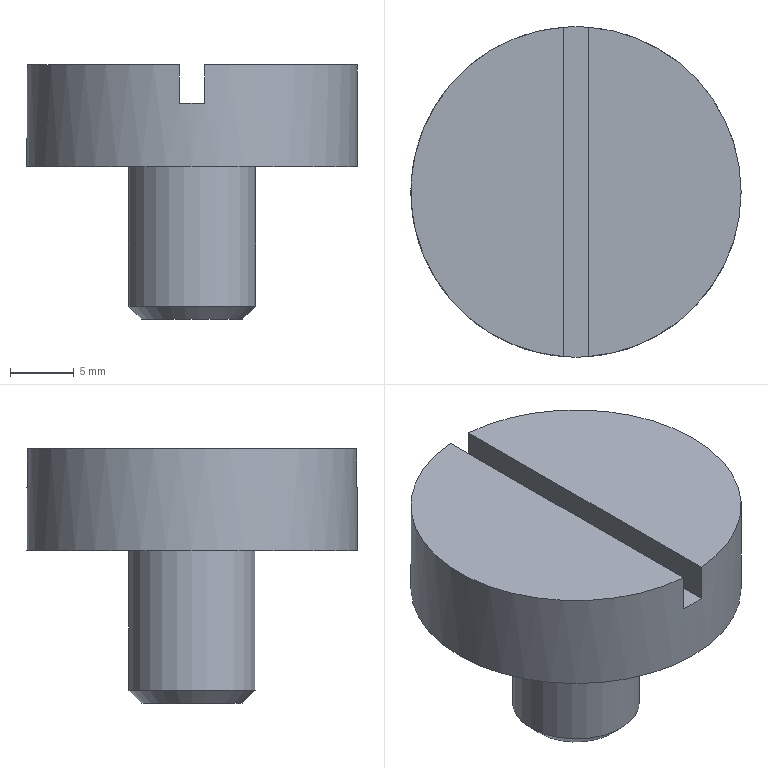Component | NX | 4 | 1 solid | 10 faces | box 26 x 26 x 20 mm | volume 5019 mm3 | plane 7 | cylinder 2 | cone 1 | commonest cylinder face diameters 26 x1 10 x1
STEP:
#1=CARTESIAN_POINT('',(0.,0.,0.));
#2=DIRECTION('',(0.,0.,1.));
#3=DIRECTION('',(1.,0.,0.));
#4=AXIS2_PLACEMENT_3D('',#1,#2,#3);
#5=CARTESIAN_POINT('',(65.,-12.961,57.));
#6=VERTEX_POINT('',#5);
#7=CARTESIAN_POINT('',(65.,12.961,57.));
#8=VERTEX_POINT('',#7);
#9=CARTESIAN_POINT('',(65.,-0.,57.));
#10=DIRECTION('',(0.,1.,0.));
#11=VECTOR('',#10,1.);
#12=LINE('',#9,#11);
#13=CARTESIAN_POINT('',(64.,-0.,57.));
#14=DIRECTION('',(-0.,0.,-1.));
#15=DIRECTION('',(1.,0.,-0.));
#16=AXIS2_PLACEMENT_3D('',#13,#14,#15);
#17=PLANE('',#16);
#18=CARTESIAN_POINT('',(1.,0.));
#19=DIRECTION('',(0.,-1.));
#20=VECTOR('',#19,1.);
#21=LINE('',#18,#20);
#22=(GEOMETRIC_REPRESENTATION_CONTEXT(2)PARAMETRIC_REPRESENTATION_CONTEXT()REPRESENTATION_CONTEXT('',''));
#23=DEFINITIONAL_REPRESENTATION('',(#21),#22);
#24=PCURVE('',#17,#23);
#25=CARTESIAN_POINT('',(65.,-29.5,54.));
#26=DIRECTION('',(-1.,0.,-0.));
#27=DIRECTION('',(0.,0.,-1.));
#28=AXIS2_PLACEMENT_3D('',#25,#26,#27);
#29=PLANE('',#28);
#30=CARTESIAN_POINT('',(-3.,-29.5));
#31=DIRECTION('',(0.,-1.));
#32=VECTOR('',#31,1.);
#33=LINE('',#30,#32);
#34=(GEOMETRIC_REPRESENTATION_CONTEXT(2)PARAMETRIC_REPRESENTATION_CONTEXT()REPRESENTATION_CONTEXT('',''));
#35=DEFINITIONAL_REPRESENTATION('',(#33),#34);
#36=PCURVE('',#29,#35);
#37=SURFACE_CURVE('',#12,(#24,#36),.PCURVE_S1.);
#38=EDGE_CURVE('',#6,#8,#37,.T.);
#39=ORIENTED_EDGE('',*,*,#38,.F.);
#40=CARTESIAN_POINT('',(77.,-0.,57.));
#41=VERTEX_POINT('',#40);
#42=CARTESIAN_POINT('',(64.,-0.,57.));
#43=DIRECTION('',(-0.,0.,-1.));
#44=DIRECTION('',(1.,0.,-0.));
#45=AXIS2_PLACEMENT_3D('',#42,#43,#44);
#46=CIRCLE('',#45,13.);
#47=CARTESIAN_POINT('',(0.,0.));
#48=DIRECTION('',(1.,0.));
#49=AXIS2_PLACEMENT_2D('',#47,#48);
#50=CIRCLE('',#49,13.);
#51=(GEOMETRIC_REPRESENTATION_CONTEXT(2)PARAMETRIC_REPRESENTATION_CONTEXT()REPRESENTATION_CONTEXT('',''));
#52=DEFINITIONAL_REPRESENTATION('',(#50),#51);
#53=PCURVE('',#17,#52);
#54=CARTESIAN_POINT('',(64.,-0.,57.));
#55=DIRECTION('',(-0.,0.,-1.));
#56=DIRECTION('',(1.,0.,-0.));
#57=AXIS2_PLACEMENT_3D('',#54,#55,#56);
#58=CYLINDRICAL_SURFACE('',#57,13.);
#59=CARTESIAN_POINT('',(-6.283,0.));
#60=DIRECTION('',(1.,0.));
#61=VECTOR('',#60,1.);
#62=LINE('',#59,#61);
#63=(GEOMETRIC_REPRESENTATION_CONTEXT(2)PARAMETRIC_REPRESENTATION_CONTEXT()REPRESENTATION_CONTEXT('',''));
#64=DEFINITIONAL_REPRESENTATION('',(#62),#63);
#65=PCURVE('',#58,#64);
#66=SURFACE_CURVE('',#46,(#53,#65),.PCURVE_S1.);
#67=EDGE_CURVE('',#41,#6,#66,.T.);
#68=ORIENTED_EDGE('',*,*,#67,.F.);
#69=CARTESIAN_POINT('',(64.,-0.,57.));
#70=DIRECTION('',(-0.,0.,-1.));
#71=DIRECTION('',(1.,0.,-0.));
#72=AXIS2_PLACEMENT_3D('',#69,#70,#71);
#73=CIRCLE('',#72,13.);
#74=CARTESIAN_POINT('',(0.,0.));
#75=DIRECTION('',(1.,0.));
#76=AXIS2_PLACEMENT_2D('',#74,#75);
#77=CIRCLE('',#76,13.);
#78=(GEOMETRIC_REPRESENTATION_CONTEXT(2)PARAMETRIC_REPRESENTATION_CONTEXT()REPRESENTATION_CONTEXT('',''));
#79=DEFINITIONAL_REPRESENTATION('',(#77),#78);
#80=PCURVE('',#17,#79);
#81=CARTESIAN_POINT('',(0.,0.));
#82=DIRECTION('',(1.,0.));
#83=VECTOR('',#82,1.);
#84=LINE('',#81,#83);
#85=(GEOMETRIC_REPRESENTATION_CONTEXT(2)PARAMETRIC_REPRESENTATION_CONTEXT()REPRESENTATION_CONTEXT('',''));
#86=DEFINITIONAL_REPRESENTATION('',(#84),#85);
#87=PCURVE('',#58,#86);
#88=SURFACE_CURVE('',#73,(#80,#87),.PCURVE_S1.);
#89=EDGE_CURVE('',#8,#41,#88,.T.);
#90=ORIENTED_EDGE('',*,*,#89,.F.);
#91=EDGE_LOOP('',(#39,#68,#90));
#92=FACE_BOUND('',#91,.T.);
#93=ADVANCED_FACE('',(#92),#17,.F.);
#94=CARTESIAN_POINT('',(63.,12.961,57.));
#95=VERTEX_POINT('',#94);
#96=CARTESIAN_POINT('',(63.,-12.961,57.));
#97=VERTEX_POINT('',#96);
#98=CARTESIAN_POINT('',(63.,-0.,57.));
#99=DIRECTION('',(0.,-1.,0.));
#100=VECTOR('',#99,1.);
#101=LINE('',#98,#100);
#102=CARTESIAN_POINT('',(64.,-0.,57.));
#103=DIRECTION('',(-0.,0.,-1.));
#104=DIRECTION('',(1.,0.,-0.));
#105=AXIS2_PLACEMENT_3D('',#102,#103,#104);
#106=PLANE('',#105);
#107=CARTESIAN_POINT('',(-1.,0.));
#108=DIRECTION('',(0.,1.));
#109=VECTOR('',#108,1.);
#110=LINE('',#107,#109);
#111=(GEOMETRIC_REPRESENTATION_CONTEXT(2)PARAMETRIC_REPRESENTATION_CONTEXT()REPRESENTATION_CONTEXT('',''));
#112=DEFINITIONAL_REPRESENTATION('',(#110),#111);
#113=PCURVE('',#106,#112);
#114=CARTESIAN_POINT('',(63.,-29.5,64.278));
#115=DIRECTION('',(1.,0.,-0.));
#116=DIRECTION('',(0.,0.,1.));
#117=AXIS2_PLACEMENT_3D('',#114,#115,#116);
#118=PLANE('',#117);
#119=CARTESIAN_POINT('',(-7.278,-29.5));
#120=DIRECTION('',(0.,1.));
#121=VECTOR('',#120,1.);
#122=LINE('',#119,#121);
#123=(GEOMETRIC_REPRESENTATION_CONTEXT(2)PARAMETRIC_REPRESENTATION_CONTEXT()REPRESENTATION_CONTEXT('',''));
#124=DEFINITIONAL_REPRESENTATION('',(#122),#123);
#125=PCURVE('',#118,#124);
#126=SURFACE_CURVE('',#101,(#113,#125),.PCURVE_S1.);
#127=EDGE_CURVE('',#95,#97,#126,.T.);
#128=ORIENTED_EDGE('',*,*,#127,.F.);
#129=CARTESIAN_POINT('',(64.,-0.,57.));
#130=DIRECTION('',(-0.,0.,-1.));
#131=DIRECTION('',(1.,0.,-0.));
#132=AXIS2_PLACEMENT_3D('',#129,#130,#131);
#133=CIRCLE('',#132,13.);
#134=CARTESIAN_POINT('',(0.,0.));
#135=DIRECTION('',(1.,0.));
#136=AXIS2_PLACEMENT_2D('',#134,#135);
#137=CIRCLE('',#136,13.);
#138=(GEOMETRIC_REPRESENTATION_CONTEXT(2)PARAMETRIC_REPRESENTATION_CONTEXT()REPRESENTATION_CONTEXT('',''));
#139=DEFINITIONAL_REPRESENTATION('',(#137),#138);
#140=PCURVE('',#106,#139);
#141=CARTESIAN_POINT('',(0.,0.));
#142=DIRECTION('',(1.,0.));
#143=VECTOR('',#142,1.);
#144=LINE('',#141,#143);
#145=(GEOMETRIC_REPRESENTATION_CONTEXT(2)PARAMETRIC_REPRESENTATION_CONTEXT()REPRESENTATION_CONTEXT('',''));
#146=DEFINITIONAL_REPRESENTATION('',(#144),#145);
#147=PCURVE('',#58,#146);
#148=SURFACE_CURVE('',#133,(#140,#147),.PCURVE_S1.);
#149=EDGE_CURVE('',#97,#95,#148,.T.);
#150=ORIENTED_EDGE('',*,*,#149,.F.);
#151=EDGE_LOOP('',(#128,#150));
#152=FACE_BOUND('',#151,.T.);
#153=ADVANCED_FACE('',(#152),#106,.F.);
#154=CARTESIAN_POINT('',(77.,-0.,49.));
#155=VERTEX_POINT('',#154);
#156=CARTESIAN_POINT('',(64.,-0.,49.));
#157=DIRECTION('',(-0.,0.,-1.));
#158=DIRECTION('',(1.,0.,-0.));
#159=AXIS2_PLACEMENT_3D('',#156,#157,#158);
#160=CIRCLE('',#159,13.);
#161=CARTESIAN_POINT('',(0.,8.));
#162=DIRECTION('',(1.,0.));
#163=VECTOR('',#162,1.);
#164=LINE('',#161,#163);
#165=(GEOMETRIC_REPRESENTATION_CONTEXT(2)PARAMETRIC_REPRESENTATION_CONTEXT()REPRESENTATION_CONTEXT('',''));
#166=DEFINITIONAL_REPRESENTATION('',(#164),#165);
#167=PCURVE('',#58,#166);
#168=CARTESIAN_POINT('',(51.,-0.,49.));
#169=DIRECTION('',(0.,0.,1.));
#170=DIRECTION('',(-1.,0.,0.));
#171=AXIS2_PLACEMENT_3D('',#168,#169,#170);
#172=PLANE('',#171);
#173=CARTESIAN_POINT('',(-26.,0.));
#174=CARTESIAN_POINT('',(-26.,22.517));
#175=CARTESIAN_POINT('',(-6.5,11.258));
#176=CARTESIAN_POINT('',(13.,0.));
#177=CARTESIAN_POINT('',(-6.5,-11.258));
#178=CARTESIAN_POINT('',(-26.,-22.517));
#179=CARTESIAN_POINT('',(-26.,0.));
#180=(BOUNDED_CURVE()B_SPLINE_CURVE(2,(#173,#174,#175,#176,#177,#178,#179),.UNSPECIFIED.,.T.,.F.)B_SPLINE_CURVE_WITH_KNOTS((1,2,2,2,2,1),(-2.094,0.,2.094,4.189,6.283,8.378),.UNSPECIFIED.)CURVE()GEOMETRIC_REPRESENTATION_ITEM()RATIONAL_B_SPLINE_CURVE((1.,0.5,1.,0.5,1.,0.5,1.))REPRESENTATION_ITEM(''));
#181=(GEOMETRIC_REPRESENTATION_CONTEXT(2)PARAMETRIC_REPRESENTATION_CONTEXT()REPRESENTATION_CONTEXT('',''));
#182=DEFINITIONAL_REPRESENTATION('',(#180),#181);
#183=PCURVE('',#172,#182);
#184=SURFACE_CURVE('',#160,(#167,#183),.PCURVE_S1.);
#185=EDGE_CURVE('',#155,#155,#184,.T.);
#186=ORIENTED_EDGE('',*,*,#185,.F.);
#187=CARTESIAN_POINT('',(77.,-0.,57.));
#188=CARTESIAN_POINT('',(77.,-0.,49.));
#189=B_SPLINE_CURVE_WITH_KNOTS('',1,(#187,#188),.UNSPECIFIED.,.F.,.F.,(2,2),(0.,8.),.PIECEWISE_BEZIER_KNOTS.);
#190=CARTESIAN_POINT('',(0.,0.));
#191=DIRECTION('',(0.,1.));
#192=VECTOR('',#191,1.);
#193=LINE('',#190,#192);
#194=(GEOMETRIC_REPRESENTATION_CONTEXT(2)PARAMETRIC_REPRESENTATION_CONTEXT()REPRESENTATION_CONTEXT('',''));
#195=DEFINITIONAL_REPRESENTATION('',(#193),#194);
#196=PCURVE('',#58,#195);
#197=CARTESIAN_POINT('',(6.283,0.));
#198=DIRECTION('',(0.,1.));
#199=VECTOR('',#198,1.);
#200=LINE('',#197,#199);
#201=(GEOMETRIC_REPRESENTATION_CONTEXT(2)PARAMETRIC_REPRESENTATION_CONTEXT()REPRESENTATION_CONTEXT('',''));
#202=DEFINITIONAL_REPRESENTATION('',(#200),#201);
#203=PCURVE('',#58,#202);
#204=SEAM_CURVE('',#189,(#196,#203),.PCURVE_S1.);
#205=EDGE_CURVE('',#41,#155,#204,.T.);
#206=ORIENTED_EDGE('',*,*,#205,.F.);
#207=ORIENTED_EDGE('',*,*,#67,.T.);
#208=CARTESIAN_POINT('',(65.,-12.961,54.));
#209=VERTEX_POINT('',#208);
#210=CARTESIAN_POINT('',(65.,-12.961,57.));
#211=DIRECTION('',(0.,0.,1.));
#212=VECTOR('',#211,1.);
#213=LINE('',#210,#212);
#214=CARTESIAN_POINT('',(1.494,0.));
#215=DIRECTION('',(0.,-1.));
#216=VECTOR('',#215,1.);
#217=LINE('',#214,#216);
#218=(GEOMETRIC_REPRESENTATION_CONTEXT(2)PARAMETRIC_REPRESENTATION_CONTEXT()REPRESENTATION_CONTEXT('',''));
#219=DEFINITIONAL_REPRESENTATION('',(#217),#218);
#220=PCURVE('',#58,#219);
#221=CARTESIAN_POINT('',(-3.,-16.539));
#222=DIRECTION('',(-1.,0.));
#223=VECTOR('',#222,1.);
#224=LINE('',#221,#223);
#225=(GEOMETRIC_REPRESENTATION_CONTEXT(2)PARAMETRIC_REPRESENTATION_CONTEXT()REPRESENTATION_CONTEXT('',''));
#226=DEFINITIONAL_REPRESENTATION('',(#224),#225);
#227=PCURVE('',#29,#226);
#228=SURFACE_CURVE('',#213,(#220,#227),.PCURVE_S1.);
#229=EDGE_CURVE('',#209,#6,#228,.T.);
#230=ORIENTED_EDGE('',*,*,#229,.F.);
#231=CARTESIAN_POINT('',(63.,-12.961,54.));
#232=VERTEX_POINT('',#231);
#233=CARTESIAN_POINT('',(64.,-0.,54.));
#234=DIRECTION('',(0.,0.,1.));
#235=DIRECTION('',(-1.,0.,0.));
#236=AXIS2_PLACEMENT_3D('',#233,#234,#235);
#237=CIRCLE('',#236,13.);
#238=CARTESIAN_POINT('',(3.142,3.));
#239=DIRECTION('',(-1.,0.));
#240=VECTOR('',#239,1.);
#241=LINE('',#238,#240);
#242=(GEOMETRIC_REPRESENTATION_CONTEXT(2)PARAMETRIC_REPRESENTATION_CONTEXT()REPRESENTATION_CONTEXT('',''));
#243=DEFINITIONAL_REPRESENTATION('',(#241),#242);
#244=PCURVE('',#58,#243);
#245=CARTESIAN_POINT('',(63.,-29.5,54.));
#246=DIRECTION('',(0.,0.,1.));
#247=DIRECTION('',(-1.,0.,0.));
#248=AXIS2_PLACEMENT_3D('',#245,#246,#247);
#249=PLANE('',#248);
#250=CARTESIAN_POINT('',(-1.,-29.5));
#251=DIRECTION('',(1.,0.));
#252=AXIS2_PLACEMENT_2D('',#250,#251);
#253=CIRCLE('',#252,13.);
#254=(GEOMETRIC_REPRESENTATION_CONTEXT(2)PARAMETRIC_REPRESENTATION_CONTEXT()REPRESENTATION_CONTEXT('',''));
#255=DEFINITIONAL_REPRESENTATION('',(#253),#254);
#256=PCURVE('',#249,#255);
#257=SURFACE_CURVE('',#237,(#244,#256),.PCURVE_S1.);
#258=EDGE_CURVE('',#232,#209,#257,.T.);
#259=ORIENTED_EDGE('',*,*,#258,.F.);
#260=CARTESIAN_POINT('',(63.,-12.961,57.));
#261=DIRECTION('',(-0.,0.,-1.));
#262=VECTOR('',#261,1.);
#263=LINE('',#260,#262);
#264=CARTESIAN_POINT('',(1.648,0.));
#265=DIRECTION('',(-0.,1.));
#266=VECTOR('',#265,1.);
#267=LINE('',#264,#266);
#268=(GEOMETRIC_REPRESENTATION_CONTEXT(2)PARAMETRIC_REPRESENTATION_CONTEXT()REPRESENTATION_CONTEXT('',''));
#269=DEFINITIONAL_REPRESENTATION('',(#267),#268);
#270=PCURVE('',#58,#269);
#271=CARTESIAN_POINT('',(-7.278,-16.539));
#272=DIRECTION('',(-1.,0.));
#273=VECTOR('',#272,1.);
#274=LINE('',#271,#273);
#275=(GEOMETRIC_REPRESENTATION_CONTEXT(2)PARAMETRIC_REPRESENTATION_CONTEXT()REPRESENTATION_CONTEXT('',''));
#276=DEFINITIONAL_REPRESENTATION('',(#274),#275);
#277=PCURVE('',#118,#276);
#278=SURFACE_CURVE('',#263,(#270,#277),.PCURVE_S1.);
#279=EDGE_CURVE('',#97,#232,#278,.T.);
#280=ORIENTED_EDGE('',*,*,#279,.F.);
#281=ORIENTED_EDGE('',*,*,#149,.T.);
#282=CARTESIAN_POINT('',(63.,12.961,54.));
#283=VERTEX_POINT('',#282);
#284=CARTESIAN_POINT('',(63.,12.961,57.));
#285=DIRECTION('',(0.,0.,1.));
#286=VECTOR('',#285,1.);
#287=LINE('',#284,#286);
#288=CARTESIAN_POINT('',(4.635,0.));
#289=DIRECTION('',(-0.,-1.));
#290=VECTOR('',#289,1.);
#291=LINE('',#288,#290);
#292=(GEOMETRIC_REPRESENTATION_CONTEXT(2)PARAMETRIC_REPRESENTATION_CONTEXT()REPRESENTATION_CONTEXT('',''));
#293=DEFINITIONAL_REPRESENTATION('',(#291),#292);
#294=PCURVE('',#58,#293);
#295=CARTESIAN_POINT('',(-7.278,-42.461));
#296=DIRECTION('',(1.,0.));
#297=VECTOR('',#296,1.);
#298=LINE('',#295,#297);
#299=(GEOMETRIC_REPRESENTATION_CONTEXT(2)PARAMETRIC_REPRESENTATION_CONTEXT()REPRESENTATION_CONTEXT('',''));
#300=DEFINITIONAL_REPRESENTATION('',(#298),#299);
#301=PCURVE('',#118,#300);
#302=SURFACE_CURVE('',#287,(#294,#301),.PCURVE_S1.);
#303=EDGE_CURVE('',#283,#95,#302,.T.);
#304=ORIENTED_EDGE('',*,*,#303,.F.);
#305=CARTESIAN_POINT('',(65.,12.961,54.));
#306=VERTEX_POINT('',#305);
#307=CARTESIAN_POINT('',(64.,-0.,54.));
#308=DIRECTION('',(0.,0.,1.));
#309=DIRECTION('',(-1.,0.,0.));
#310=AXIS2_PLACEMENT_3D('',#307,#308,#309);
#311=CIRCLE('',#310,13.);
#312=CARTESIAN_POINT('',(9.425,3.));
#313=DIRECTION('',(-1.,0.));
#314=VECTOR('',#313,1.);
#315=LINE('',#312,#314);
#316=(GEOMETRIC_REPRESENTATION_CONTEXT(2)PARAMETRIC_REPRESENTATION_CONTEXT()REPRESENTATION_CONTEXT('',''));
#317=DEFINITIONAL_REPRESENTATION('',(#315),#316);
#318=PCURVE('',#58,#317);
#319=CARTESIAN_POINT('',(-1.,-29.5));
#320=DIRECTION('',(1.,0.));
#321=AXIS2_PLACEMENT_2D('',#319,#320);
#322=CIRCLE('',#321,13.);
#323=(GEOMETRIC_REPRESENTATION_CONTEXT(2)PARAMETRIC_REPRESENTATION_CONTEXT()REPRESENTATION_CONTEXT('',''));
#324=DEFINITIONAL_REPRESENTATION('',(#322),#323);
#325=PCURVE('',#249,#324);
#326=SURFACE_CURVE('',#311,(#318,#325),.PCURVE_S1.);
#327=EDGE_CURVE('',#306,#283,#326,.T.);
#328=ORIENTED_EDGE('',*,*,#327,.F.);
#329=CARTESIAN_POINT('',(65.,12.961,57.));
#330=DIRECTION('',(-0.,0.,-1.));
#331=VECTOR('',#330,1.);
#332=LINE('',#329,#331);
#333=CARTESIAN_POINT('',(4.789,0.));
#334=DIRECTION('',(0.,1.));
#335=VECTOR('',#334,1.);
#336=LINE('',#333,#335);
#337=(GEOMETRIC_REPRESENTATION_CONTEXT(2)PARAMETRIC_REPRESENTATION_CONTEXT()REPRESENTATION_CONTEXT('',''));
#338=DEFINITIONAL_REPRESENTATION('',(#336),#337);
#339=PCURVE('',#58,#338);
#340=CARTESIAN_POINT('',(-3.,-42.461));
#341=DIRECTION('',(1.,0.));
#342=VECTOR('',#341,1.);
#343=LINE('',#340,#342);
#344=(GEOMETRIC_REPRESENTATION_CONTEXT(2)PARAMETRIC_REPRESENTATION_CONTEXT()REPRESENTATION_CONTEXT('',''));
#345=DEFINITIONAL_REPRESENTATION('',(#343),#344);
#346=PCURVE('',#29,#345);
#347=SURFACE_CURVE('',#332,(#339,#346),.PCURVE_S1.);
#348=EDGE_CURVE('',#8,#306,#347,.T.);
#349=ORIENTED_EDGE('',*,*,#348,.F.);
#350=ORIENTED_EDGE('',*,*,#89,.T.);
#351=ORIENTED_EDGE('',*,*,#205,.T.);
#352=EDGE_LOOP('',(#186,#206,#207,#230,#259,#280,#281,#304,#328,#349,#350,#351));
#353=FACE_BOUND('',#352,.T.);
#354=ADVANCED_FACE('',(#353),#58,.T.);
#355=CARTESIAN_POINT('',(60.,-0.,37.));
#356=VERTEX_POINT('',#355);
#357=CARTESIAN_POINT('',(64.,-0.,37.));
#358=DIRECTION('',(-0.,0.,-1.));
#359=DIRECTION('',(-1.,0.,0.));
#360=AXIS2_PLACEMENT_3D('',#357,#358,#359);
#361=CIRCLE('',#360,4.);
#362=CARTESIAN_POINT('',(59.,-0.,37.));
#363=DIRECTION('',(0.,0.,1.));
#364=DIRECTION('',(-1.,0.,0.));
#365=AXIS2_PLACEMENT_3D('',#362,#363,#364);
#366=PLANE('',#365);
#367=CARTESIAN_POINT('',(-1.,0.));
#368=CARTESIAN_POINT('',(-1.,-6.928));
#369=CARTESIAN_POINT('',(-7.,-3.464));
#370=CARTESIAN_POINT('',(-13.,-0.));
#371=CARTESIAN_POINT('',(-7.,3.464));
#372=CARTESIAN_POINT('',(-1.,6.928));
#373=CARTESIAN_POINT('',(-1.,0.));
#374=(BOUNDED_CURVE()B_SPLINE_CURVE(2,(#367,#368,#369,#370,#371,#372,#373),.UNSPECIFIED.,.T.,.F.)B_SPLINE_CURVE_WITH_KNOTS((1,2,2,2,2,1),(-2.094,0.,2.094,4.189,6.283,8.378),.UNSPECIFIED.)CURVE()GEOMETRIC_REPRESENTATION_ITEM()RATIONAL_B_SPLINE_CURVE((1.,0.5,1.,0.5,1.,0.5,1.))REPRESENTATION_ITEM(''));
#375=(GEOMETRIC_REPRESENTATION_CONTEXT(2)PARAMETRIC_REPRESENTATION_CONTEXT()REPRESENTATION_CONTEXT('',''));
#376=DEFINITIONAL_REPRESENTATION('',(#374),#375);
#377=PCURVE('',#366,#376);
#378=CARTESIAN_POINT('',(64.,-0.,37.));
#379=DIRECTION('',(0.,0.,1.));
#380=DIRECTION('',(-1.,0.,0.));
#381=AXIS2_PLACEMENT_3D('',#378,#379,#380);
#382=CONICAL_SURFACE('',#381,4.,0.7854);
#383=CARTESIAN_POINT('',(6.283,-0.));
#384=DIRECTION('',(-1.,0.));
#385=VECTOR('',#384,1.);
#386=LINE('',#383,#385);
#387=(GEOMETRIC_REPRESENTATION_CONTEXT(2)PARAMETRIC_REPRESENTATION_CONTEXT()REPRESENTATION_CONTEXT('',''));
#388=DEFINITIONAL_REPRESENTATION('',(#386),#387);
#389=PCURVE('',#382,#388);
#390=SURFACE_CURVE('',#361,(#377,#389),.PCURVE_S1.);
#391=EDGE_CURVE('',#356,#356,#390,.T.);
#392=ORIENTED_EDGE('',*,*,#391,.T.);
#393=EDGE_LOOP('',(#392));
#394=FACE_BOUND('',#393,.T.);
#395=ADVANCED_FACE('',(#394),#366,.F.);
#396=CARTESIAN_POINT('',(69.,-0.,49.));
#397=VERTEX_POINT('',#396);
#398=CARTESIAN_POINT('',(64.,-0.,49.));
#399=DIRECTION('',(-0.,0.,-1.));
#400=DIRECTION('',(1.,0.,-0.));
#401=AXIS2_PLACEMENT_3D('',#398,#399,#400);
#402=CIRCLE('',#401,5.);
#403=CARTESIAN_POINT('',(-18.,0.));
#404=CARTESIAN_POINT('',(-18.,8.66));
#405=CARTESIAN_POINT('',(-10.5,4.33));
#406=CARTESIAN_POINT('',(-3.,0.));
#407=CARTESIAN_POINT('',(-10.5,-4.33));
#408=CARTESIAN_POINT('',(-18.,-8.66));
#409=CARTESIAN_POINT('',(-18.,0.));
#410=(BOUNDED_CURVE()B_SPLINE_CURVE(2,(#403,#404,#405,#406,#407,#408,#409),.UNSPECIFIED.,.T.,.F.)B_SPLINE_CURVE_WITH_KNOTS((1,2,2,2,2,1),(-2.094,0.,2.094,4.189,6.283,8.378),.UNSPECIFIED.)CURVE()GEOMETRIC_REPRESENTATION_ITEM()RATIONAL_B_SPLINE_CURVE((1.,0.5,1.,0.5,1.,0.5,1.))REPRESENTATION_ITEM(''));
#411=(GEOMETRIC_REPRESENTATION_CONTEXT(2)PARAMETRIC_REPRESENTATION_CONTEXT()REPRESENTATION_CONTEXT('',''));
#412=DEFINITIONAL_REPRESENTATION('',(#410),#411);
#413=PCURVE('',#172,#412);
#414=CARTESIAN_POINT('',(64.,-0.,57.));
#415=DIRECTION('',(-0.,0.,-1.));
#416=DIRECTION('',(1.,0.,-0.));
#417=AXIS2_PLACEMENT_3D('',#414,#415,#416);
#418=CYLINDRICAL_SURFACE('',#417,5.);
#419=CARTESIAN_POINT('',(0.,8.));
#420=DIRECTION('',(1.,0.));
#421=VECTOR('',#420,1.);
#422=LINE('',#419,#421);
#423=(GEOMETRIC_REPRESENTATION_CONTEXT(2)PARAMETRIC_REPRESENTATION_CONTEXT()REPRESENTATION_CONTEXT('',''));
#424=DEFINITIONAL_REPRESENTATION('',(#422),#423);
#425=PCURVE('',#418,#424);
#426=SURFACE_CURVE('',#402,(#413,#425),.PCURVE_S1.);
#427=EDGE_CURVE('',#397,#397,#426,.T.);
#428=ORIENTED_EDGE('',*,*,#427,.F.);
#429=EDGE_LOOP('',(#428));
#430=FACE_BOUND('',#429,.T.);
#431=ORIENTED_EDGE('',*,*,#185,.T.);
#432=EDGE_LOOP('',(#431));
#433=FACE_BOUND('',#432,.T.);
#434=ADVANCED_FACE('',(#430,#433),#172,.F.);
#435=CARTESIAN_POINT('',(59.,-0.,38.));
#436=VERTEX_POINT('',#435);
#437=CARTESIAN_POINT('',(69.,-0.,38.));
#438=VERTEX_POINT('',#437);
#439=CARTESIAN_POINT('',(64.,-0.,38.));
#440=DIRECTION('',(0.,0.,1.));
#441=DIRECTION('',(-1.,0.,0.));
#442=AXIS2_PLACEMENT_3D('',#439,#440,#441);
#443=CIRCLE('',#442,5.);
#444=CARTESIAN_POINT('',(3.142,19.));
#445=DIRECTION('',(-1.,0.));
#446=VECTOR('',#445,1.);
#447=LINE('',#444,#446);
#448=(GEOMETRIC_REPRESENTATION_CONTEXT(2)PARAMETRIC_REPRESENTATION_CONTEXT()REPRESENTATION_CONTEXT('',''));
#449=DEFINITIONAL_REPRESENTATION('',(#447),#448);
#450=PCURVE('',#418,#449);
#451=CARTESIAN_POINT('',(0.,1.));
#452=DIRECTION('',(1.,0.));
#453=VECTOR('',#452,1.);
#454=LINE('',#451,#453);
#455=(GEOMETRIC_REPRESENTATION_CONTEXT(2)PARAMETRIC_REPRESENTATION_CONTEXT()REPRESENTATION_CONTEXT('',''));
#456=DEFINITIONAL_REPRESENTATION('',(#454),#455);
#457=PCURVE('',#382,#456);
#458=SURFACE_CURVE('',#443,(#450,#457),.PCURVE_S1.);
#459=EDGE_CURVE('',#436,#438,#458,.T.);
#460=ORIENTED_EDGE('',*,*,#459,.T.);
#461=CARTESIAN_POINT('',(69.,-0.,49.));
#462=CARTESIAN_POINT('',(69.,-0.,38.));
#463=B_SPLINE_CURVE_WITH_KNOTS('',1,(#461,#462),.UNSPECIFIED.,.F.,.F.,(2,2),(8.,19.),.PIECEWISE_BEZIER_KNOTS.);
#464=CARTESIAN_POINT('',(0.,0.));
#465=DIRECTION('',(0.,1.));
#466=VECTOR('',#465,1.);
#467=LINE('',#464,#466);
#468=(GEOMETRIC_REPRESENTATION_CONTEXT(2)PARAMETRIC_REPRESENTATION_CONTEXT()REPRESENTATION_CONTEXT('',''));
#469=DEFINITIONAL_REPRESENTATION('',(#467),#468);
#470=PCURVE('',#418,#469);
#471=CARTESIAN_POINT('',(6.283,0.));
#472=DIRECTION('',(0.,1.));
#473=VECTOR('',#472,1.);
#474=LINE('',#471,#473);
#475=(GEOMETRIC_REPRESENTATION_CONTEXT(2)PARAMETRIC_REPRESENTATION_CONTEXT()REPRESENTATION_CONTEXT('',''));
#476=DEFINITIONAL_REPRESENTATION('',(#474),#475);
#477=PCURVE('',#418,#476);
#478=SEAM_CURVE('',#463,(#470,#477),.PCURVE_S1.);
#479=EDGE_CURVE('',#397,#438,#478,.T.);
#480=ORIENTED_EDGE('',*,*,#479,.F.);
#481=ORIENTED_EDGE('',*,*,#427,.T.);
#482=ORIENTED_EDGE('',*,*,#479,.T.);
#483=CARTESIAN_POINT('',(64.,-0.,38.));
#484=DIRECTION('',(0.,0.,1.));
#485=DIRECTION('',(-1.,0.,0.));
#486=AXIS2_PLACEMENT_3D('',#483,#484,#485);
#487=CIRCLE('',#486,5.);
#488=CARTESIAN_POINT('',(9.425,19.));
#489=DIRECTION('',(-1.,0.));
#490=VECTOR('',#489,1.);
#491=LINE('',#488,#490);
#492=(GEOMETRIC_REPRESENTATION_CONTEXT(2)PARAMETRIC_REPRESENTATION_CONTEXT()REPRESENTATION_CONTEXT('',''));
#493=DEFINITIONAL_REPRESENTATION('',(#491),#492);
#494=PCURVE('',#418,#493);
#495=CARTESIAN_POINT('',(0.,1.));
#496=DIRECTION('',(1.,-0.));
#497=VECTOR('',#496,1.);
#498=LINE('',#495,#497);
#499=(GEOMETRIC_REPRESENTATION_CONTEXT(2)PARAMETRIC_REPRESENTATION_CONTEXT()REPRESENTATION_CONTEXT('',''));
#500=DEFINITIONAL_REPRESENTATION('',(#498),#499);
#501=PCURVE('',#382,#500);
#502=SURFACE_CURVE('',#487,(#494,#501),.PCURVE_S1.);
#503=EDGE_CURVE('',#438,#436,#502,.T.);
#504=ORIENTED_EDGE('',*,*,#503,.T.);
#505=EDGE_LOOP('',(#460,#480,#481,#482,#504));
#506=FACE_BOUND('',#505,.T.);
#507=ADVANCED_FACE('',(#506),#418,.T.);
#508=ORIENTED_EDGE('',*,*,#258,.T.);
#509=CARTESIAN_POINT('',(65.,-29.5,54.));
#510=DIRECTION('',(0.,-1.,0.));
#511=VECTOR('',#510,1.);
#512=LINE('',#509,#511);
#513=CARTESIAN_POINT('',(-2.,0.));
#514=DIRECTION('',(0.,1.));
#515=VECTOR('',#514,1.);
#516=LINE('',#513,#515);
#517=(GEOMETRIC_REPRESENTATION_CONTEXT(2)PARAMETRIC_REPRESENTATION_CONTEXT()REPRESENTATION_CONTEXT('',''));
#518=DEFINITIONAL_REPRESENTATION('',(#516),#517);
#519=PCURVE('',#249,#518);
#520=CARTESIAN_POINT('',(0.,0.));
#521=DIRECTION('',(0.,1.));
#522=VECTOR('',#521,1.);
#523=LINE('',#520,#522);
#524=(GEOMETRIC_REPRESENTATION_CONTEXT(2)PARAMETRIC_REPRESENTATION_CONTEXT()REPRESENTATION_CONTEXT('',''));
#525=DEFINITIONAL_REPRESENTATION('',(#523),#524);
#526=PCURVE('',#29,#525);
#527=SURFACE_CURVE('',#512,(#519,#526),.PCURVE_S1.);
#528=EDGE_CURVE('',#306,#209,#527,.T.);
#529=ORIENTED_EDGE('',*,*,#528,.F.);
#530=ORIENTED_EDGE('',*,*,#327,.T.);
#531=CARTESIAN_POINT('',(63.,-29.5,54.));
#532=DIRECTION('',(0.,-1.,0.));
#533=VECTOR('',#532,1.);
#534=LINE('',#531,#533);
#535=CARTESIAN_POINT('',(0.,0.));
#536=DIRECTION('',(0.,1.));
#537=VECTOR('',#536,1.);
#538=LINE('',#535,#537);
#539=(GEOMETRIC_REPRESENTATION_CONTEXT(2)PARAMETRIC_REPRESENTATION_CONTEXT()REPRESENTATION_CONTEXT('',''));
#540=DEFINITIONAL_REPRESENTATION('',(#538),#539);
#541=PCURVE('',#249,#540);
#542=CARTESIAN_POINT('',(-10.278,0.));
#543=DIRECTION('',(0.,1.));
#544=VECTOR('',#543,1.);
#545=LINE('',#542,#544);
#546=(GEOMETRIC_REPRESENTATION_CONTEXT(2)PARAMETRIC_REPRESENTATION_CONTEXT()REPRESENTATION_CONTEXT('',''));
#547=DEFINITIONAL_REPRESENTATION('',(#545),#546);
#548=PCURVE('',#118,#547);
#549=SURFACE_CURVE('',#534,(#541,#548),.PCURVE_S1.);
#550=EDGE_CURVE('',#283,#232,#549,.T.);
#551=ORIENTED_EDGE('',*,*,#550,.T.);
#552=EDGE_LOOP('',(#508,#529,#530,#551));
#553=FACE_BOUND('',#552,.T.);
#554=ADVANCED_FACE('',(#553),#249,.T.);
#555=ORIENTED_EDGE('',*,*,#348,.T.);
#556=ORIENTED_EDGE('',*,*,#528,.T.);
#557=ORIENTED_EDGE('',*,*,#229,.T.);
#558=ORIENTED_EDGE('',*,*,#38,.T.);
#559=EDGE_LOOP('',(#555,#556,#557,#558));
#560=FACE_BOUND('',#559,.T.);
#561=ADVANCED_FACE('',(#560),#29,.T.);
#562=ORIENTED_EDGE('',*,*,#279,.T.);
#563=ORIENTED_EDGE('',*,*,#550,.F.);
#564=ORIENTED_EDGE('',*,*,#303,.T.);
#565=ORIENTED_EDGE('',*,*,#127,.T.);
#566=EDGE_LOOP('',(#562,#563,#564,#565));
#567=FACE_BOUND('',#566,.T.);
#568=ADVANCED_FACE('',(#567),#118,.T.);
#569=ORIENTED_EDGE('',*,*,#459,.F.);
#570=CARTESIAN_POINT('',(60.,-0.,37.));
#571=CARTESIAN_POINT('',(59.,-0.,38.));
#572=B_SPLINE_CURVE_WITH_KNOTS('',1,(#570,#571),.UNSPECIFIED.,.F.,.F.,(2,2),(-0.,1.414),.PIECEWISE_BEZIER_KNOTS.);
#573=CARTESIAN_POINT('',(0.,0.));
#574=DIRECTION('',(0.,1.));
#575=VECTOR('',#574,1.);
#576=LINE('',#573,#575);
#577=(GEOMETRIC_REPRESENTATION_CONTEXT(2)PARAMETRIC_REPRESENTATION_CONTEXT()REPRESENTATION_CONTEXT('',''));
#578=DEFINITIONAL_REPRESENTATION('',(#576),#577);
#579=PCURVE('',#382,#578);
#580=CARTESIAN_POINT('',(6.283,0.));
#581=DIRECTION('',(0.,1.));
#582=VECTOR('',#581,1.);
#583=LINE('',#580,#582);
#584=(GEOMETRIC_REPRESENTATION_CONTEXT(2)PARAMETRIC_REPRESENTATION_CONTEXT()REPRESENTATION_CONTEXT('',''));
#585=DEFINITIONAL_REPRESENTATION('',(#583),#584);
#586=PCURVE('',#382,#585);
#587=SEAM_CURVE('',#572,(#579,#586),.PCURVE_S1.);
#588=EDGE_CURVE('',#356,#436,#587,.T.);
#589=ORIENTED_EDGE('',*,*,#588,.F.);
#590=ORIENTED_EDGE('',*,*,#391,.F.);
#591=ORIENTED_EDGE('',*,*,#588,.T.);
#592=ORIENTED_EDGE('',*,*,#503,.F.);
#593=EDGE_LOOP('',(#569,#589,#590,#591,#592));
#594=FACE_BOUND('',#593,.T.);
#595=ADVANCED_FACE('',(#594),#382,.T.);
#596=CLOSED_SHELL('',(#93,#153,#354,#395,#434,#507,#554,#561,#568,#595));
#597=MANIFOLD_SOLID_BREP('',#596);
#598=(LENGTH_UNIT()NAMED_UNIT(*)SI_UNIT(.MILLI.,.METRE.));
#599=UNCERTAINTY_MEASURE_WITH_UNIT(LENGTH_MEASURE(0.000002),#598,'','');
#600=(NAMED_UNIT(*)PLANE_ANGLE_UNIT()SI_UNIT($,.RADIAN.));
#601=(NAMED_UNIT(*)SI_UNIT($,.STERADIAN.)SOLID_ANGLE_UNIT());
#602=(GEOMETRIC_REPRESENTATION_CONTEXT(3)GLOBAL_UNCERTAINTY_ASSIGNED_CONTEXT((#599))GLOBAL_UNIT_ASSIGNED_CONTEXT((#598,#600,#601))REPRESENTATION_CONTEXT('',''));
#603=ADVANCED_BREP_SHAPE_REPRESENTATION('',(#4,#597),#602);